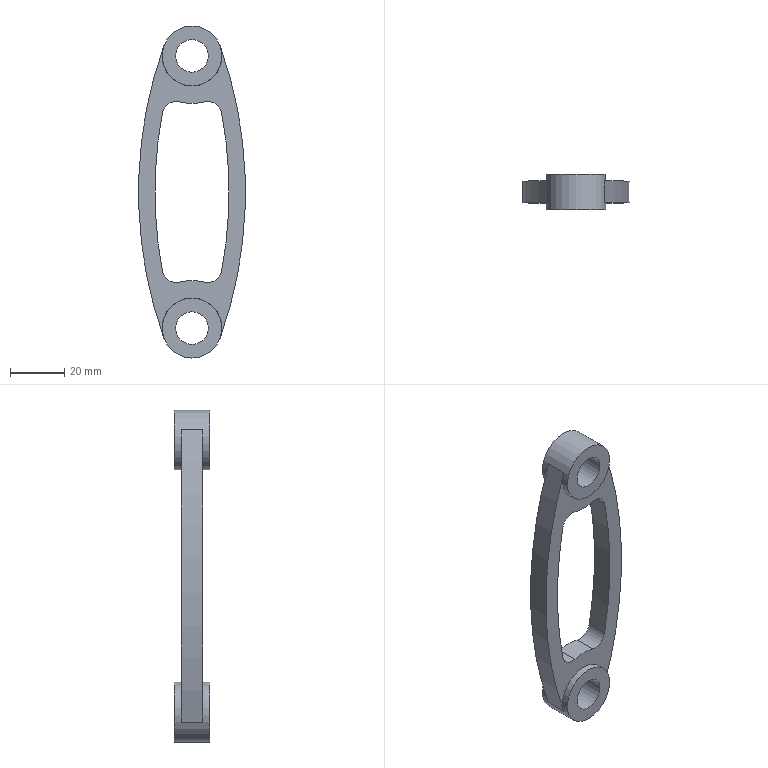Component | NX | CONNECTING_ROD | 1 solid | 20 faces | volume 18071 mm3 | cylinder 14 | plane 6 | commonest cylinder face diameters 10 x4 35 x2 308 x2 22 x2 320 x2 12 x2